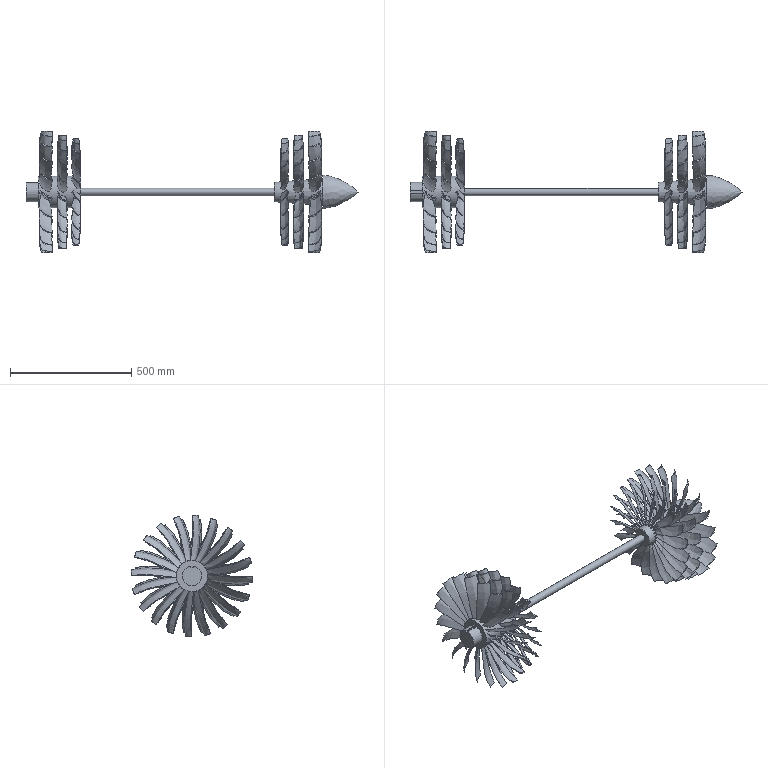Component | NX | SHAFT_WITH_BLADES | 1 solid | 373 faces | volume 8285849 mm3 | spline 241 | plane 128 | cylinder 3 | cone 1 | commonest cylinder face diameters 130 x1 80 x1 30 x1